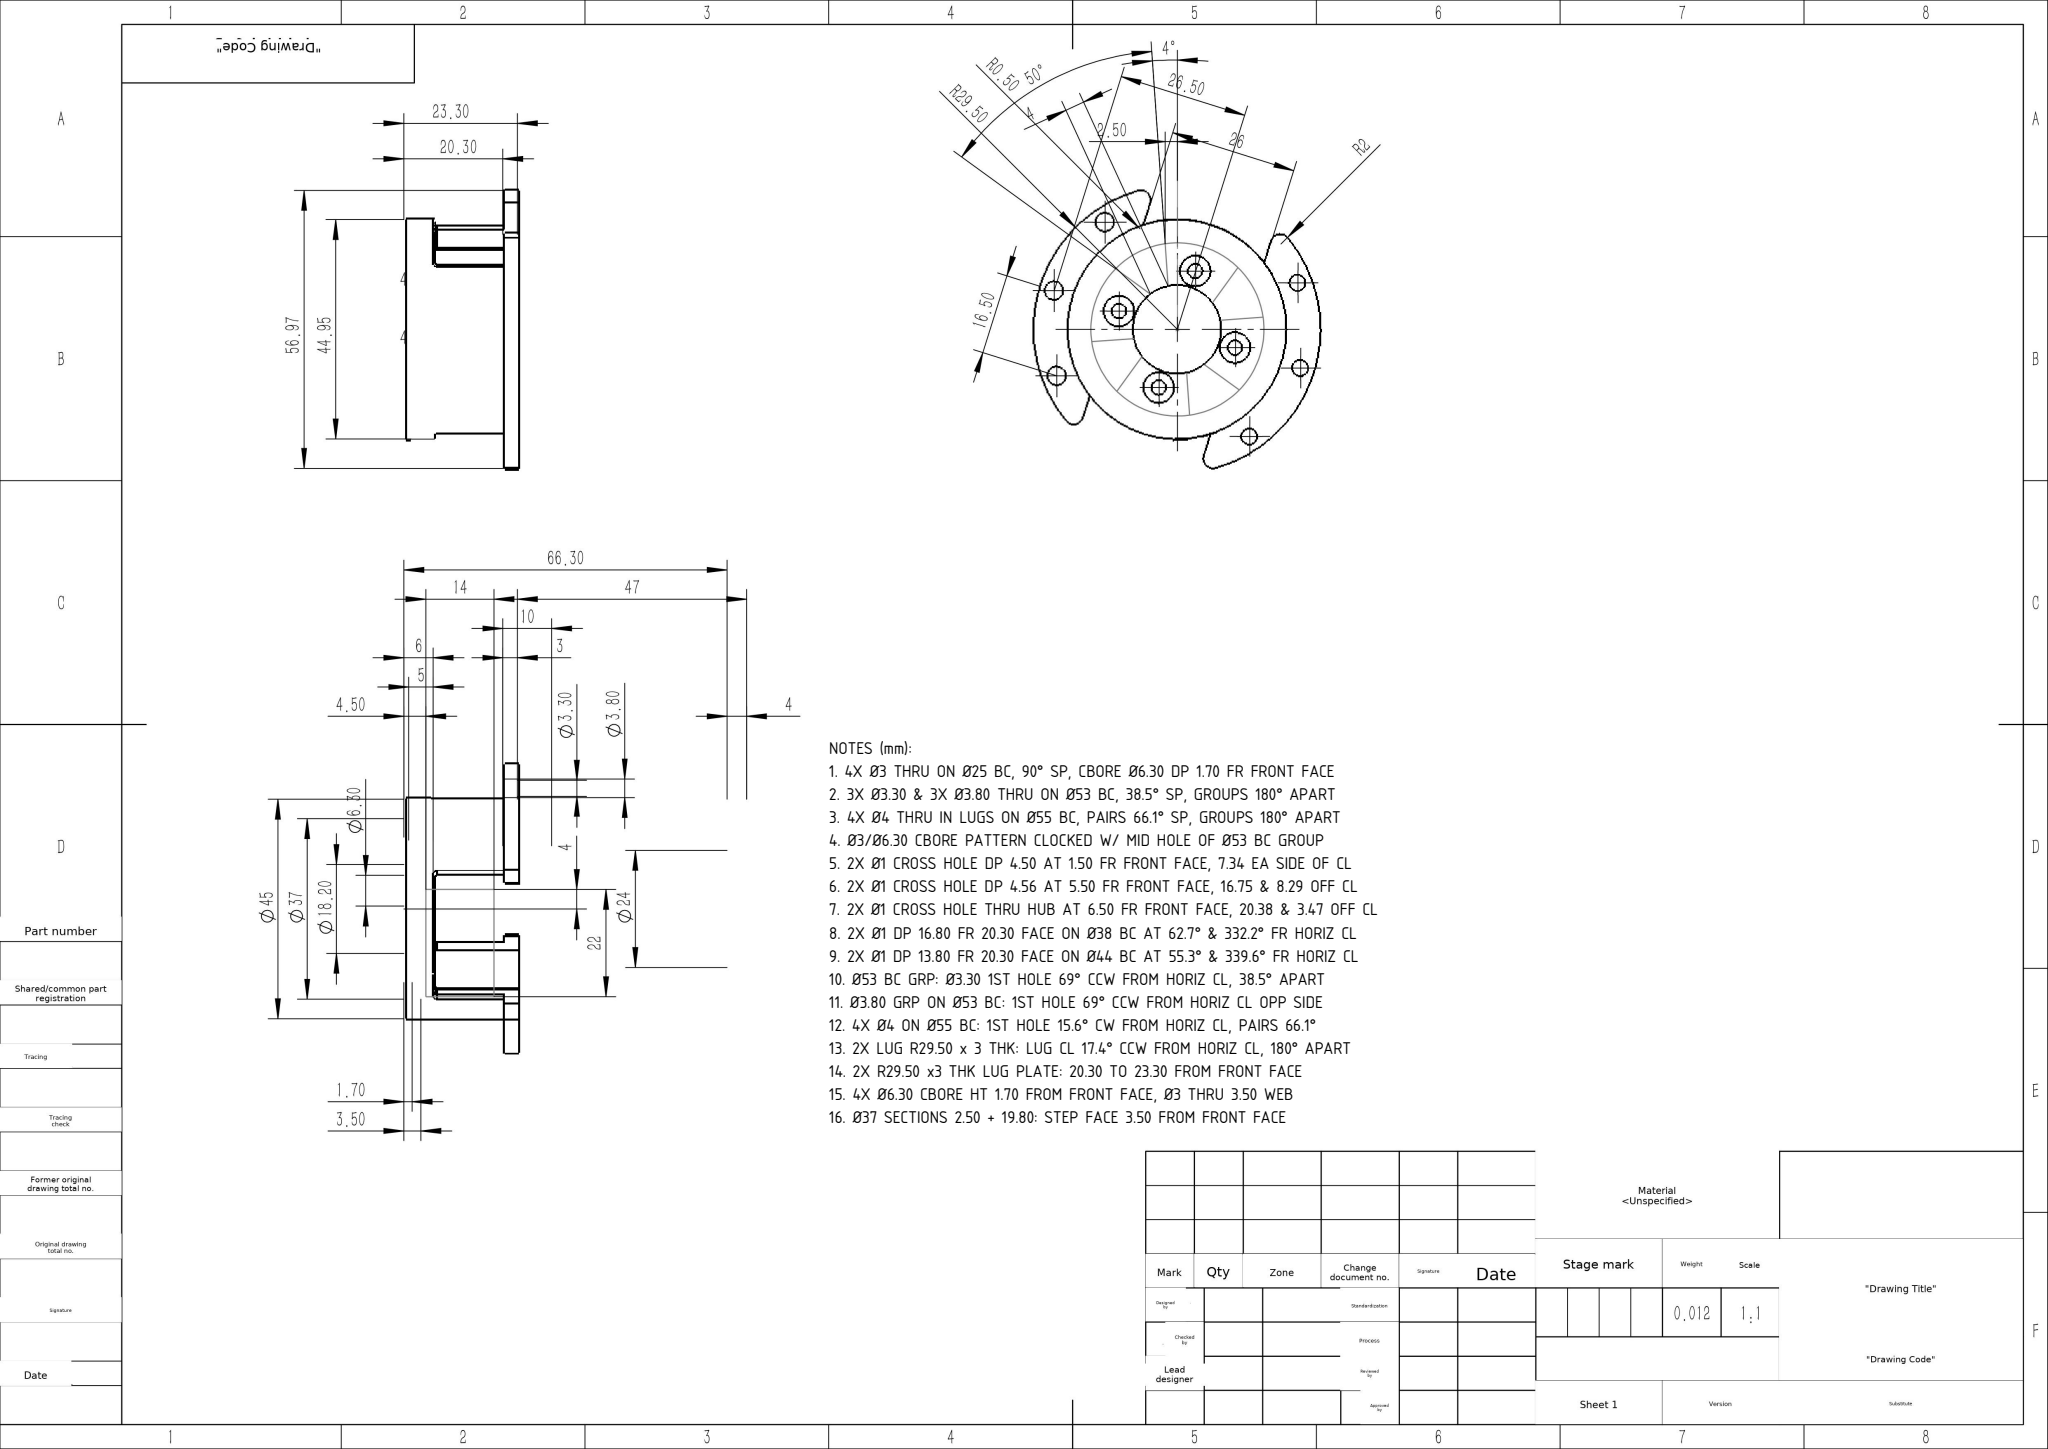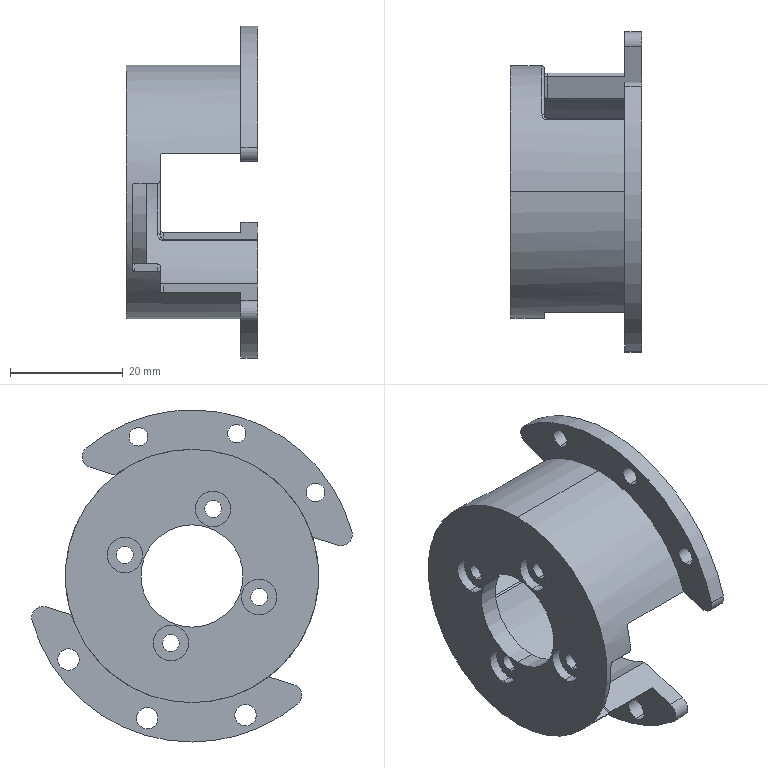Part | SolidWorks | mm | 1 solid | 83 faces | box 23.3 x 56.97 x 59 mm | volume 12419 mm3 | cylinder 57 | plane 20 | spline 4 | torus 2 | commonest cylinder face diameters 1 x13 6.3 x8 3 x8 3.8 x6 3.3 x6 4 x5 37 x4 59 x3
Drawing notes:
4X Ø3 THRU ON Ø25 BC, 90° SP, CBORE Ø6.30 DP 1.70 FR FRONT FACE | from the solid: Ø3.0 x-holes (16.56,25.75),(24.74,41.43),(32.23,17.57),(40.41,33.25), R12.50 fr axis (28.49,29.5) => Ø25 BC, 90° SP; Ø6.3 cbores same centres lg 1.7, planes x=0/1.7; Ø3 lg 1.8 thru 3.5 web
3X Ø3.30 & 3X Ø3.80 THRU ON Ø53 BC, 38.5° SP, GROUPS 180° APART | from the solid: Ø3.3 at (6.53,44.34),(20.54,54.78),(38.01,54.23); Ø3.8 at (18.96,4.77),(36.43,4.22),(50.44,14.66); all R26.50 => Ø53 BC; angles 145.95/107.46/68.95 and 325.93/287.44/249.07
4X Ø4 THRU IN LUGS ON Ø55 BC, PAIRS 66.1° SP, GROUPS 180° APART | from the solid: Ø4 holes (2.0,36.9),(10.99,8.28),(45.98,50.72),(54.97,22.1); R27.50 fr axis => Ø55 BC; angles 164.39/230.49 and 344.39/50.49
Ø3/Ø6.30 CBORE PATTERN CLOCKED W/ MID HOLE OF Ø53 BC GROUP | from the solid: Ø3 CB hole at 107.45° coincides with mid Ø3.30 hole (20.54,54.78) at 107.46°; Ø55 lug holes at 50.5/164.4/230.5/344.4°
2X Ø1 CROSS HOLE DP 4.50 AT 1.50 FR FRONT FACE, 7.34 EA SIDE OF CL | from the solid: Ø1 y-axis cyls at x=1.5, z=22.16 & 36.84, lg 4.5; ±7.34 fr axis z=29.5
2X Ø1 CROSS HOLE DP 4.56 AT 5.50 FR FRONT FACE, 16.75 & 8.29 OFF CL | from the solid: Ø1 y-axis cyls at x=5.5, z=12.75 & 37.79, lg 4.56; offsets 16.75 and 8.29 fr axis z=29.5
2X Ø1 CROSS HOLE THRU HUB AT 6.50 FR FRONT FACE, 20.38 & 3.47 OFF CL | from the solid: Ø1 y-axis cyls at x=6.5, z=9.12 & 32.97, two segments each (4.67 + 5.44) thru both walls; offsets 20.38 and 3.47 fr axis z=29.5
2X Ø1 DP 16.80 FR 20.30 FACE ON Ø38 BC AT 62.7° & 332.2° FR HORIZ CL | from the solid: Ø1 x-cyls (37.19,46.39) & (45.29,20.63) lg 16.8; R19.0 fr axis => Ø38 BC; angles 62.74° and 332.17°
2X Ø1 DP 13.80 FR 20.30 FACE ON Ø44 BC AT 55.3° & 339.6° FR HORIZ CL | from the solid: Ø1 x-cyls (41.01,47.59) & (49.10,21.83) lg 13.8; R22.0 fr axis => Ø44 BC; angles 55.30° and 339.58°
Ø53 BC GRP: Ø3.30 1ST HOLE 69° CCW FROM HORIZ CL, 38.5° APART | from the solid: Ø3.30 holes at (y,z) (6.53,44.34),(20.54,54.78),(38.01,54.23) about ctr (28.49,29.5): R26.50, angles 145.95°/107.47°/68.95° from +Y horiz CL
Ø3.80 GRP ON Ø53 BC: 1ST HOLE 69° CCW FROM HORIZ CL OPP SIDE | from the solid: Ø3.80 holes (18.96,4.77),(36.43,4.22),(50.44,14.66): R26.50, angles 248.93°/287.45°/325.94° = Ø3.30 grp +180°
4X Ø4 ON Ø55 BC: 1ST HOLE 15.6° CW FROM HORIZ CL, PAIRS 66.1° | from the solid: Ø4 holes (2.0,36.9),(10.99,8.28),(45.98,50.72),(54.97,22.1): R27.50, angles -15.61°/50.49°/164.40°/230.49°
2X LUG R29.50 x 3 THK: LUG CL 17.4° CCW FROM HORIZ CL, 180° APART | from the solid: Ø59 cyl x 3.0 lg at ctr (28.49,29.5); lug hole pair bisectors at 17.44° and 197.44°
2X R29.50 x3 THK LUG PLATE: 20.30 TO 23.30 FROM FRONT FACE | from the solid: Ø59 cyl len 3.0 between x-planes 20.30 and 23.30; bbox x=23.3; Ø45 body len 20.3 from x=0
4X Ø6.30 CBORE HT 1.70 FROM FRONT FACE, Ø3 THRU 3.50 WEB | from the solid: Ø6.3 cyls len 1.7 at r=12.5 BC, coaxial Ø3 cyls len 1.8; x-planes 0 / 1.7 / 3.5
Ø37 SECTIONS 2.50 + 19.80: STEP FACE 3.50 FROM FRONT FACE | from the solid: Ø37 len 2.5 (x 1.00-3.50) and Ø37 len 19.8 (x 3.50-23.30); planes x=1.0, 3.5, 23.3